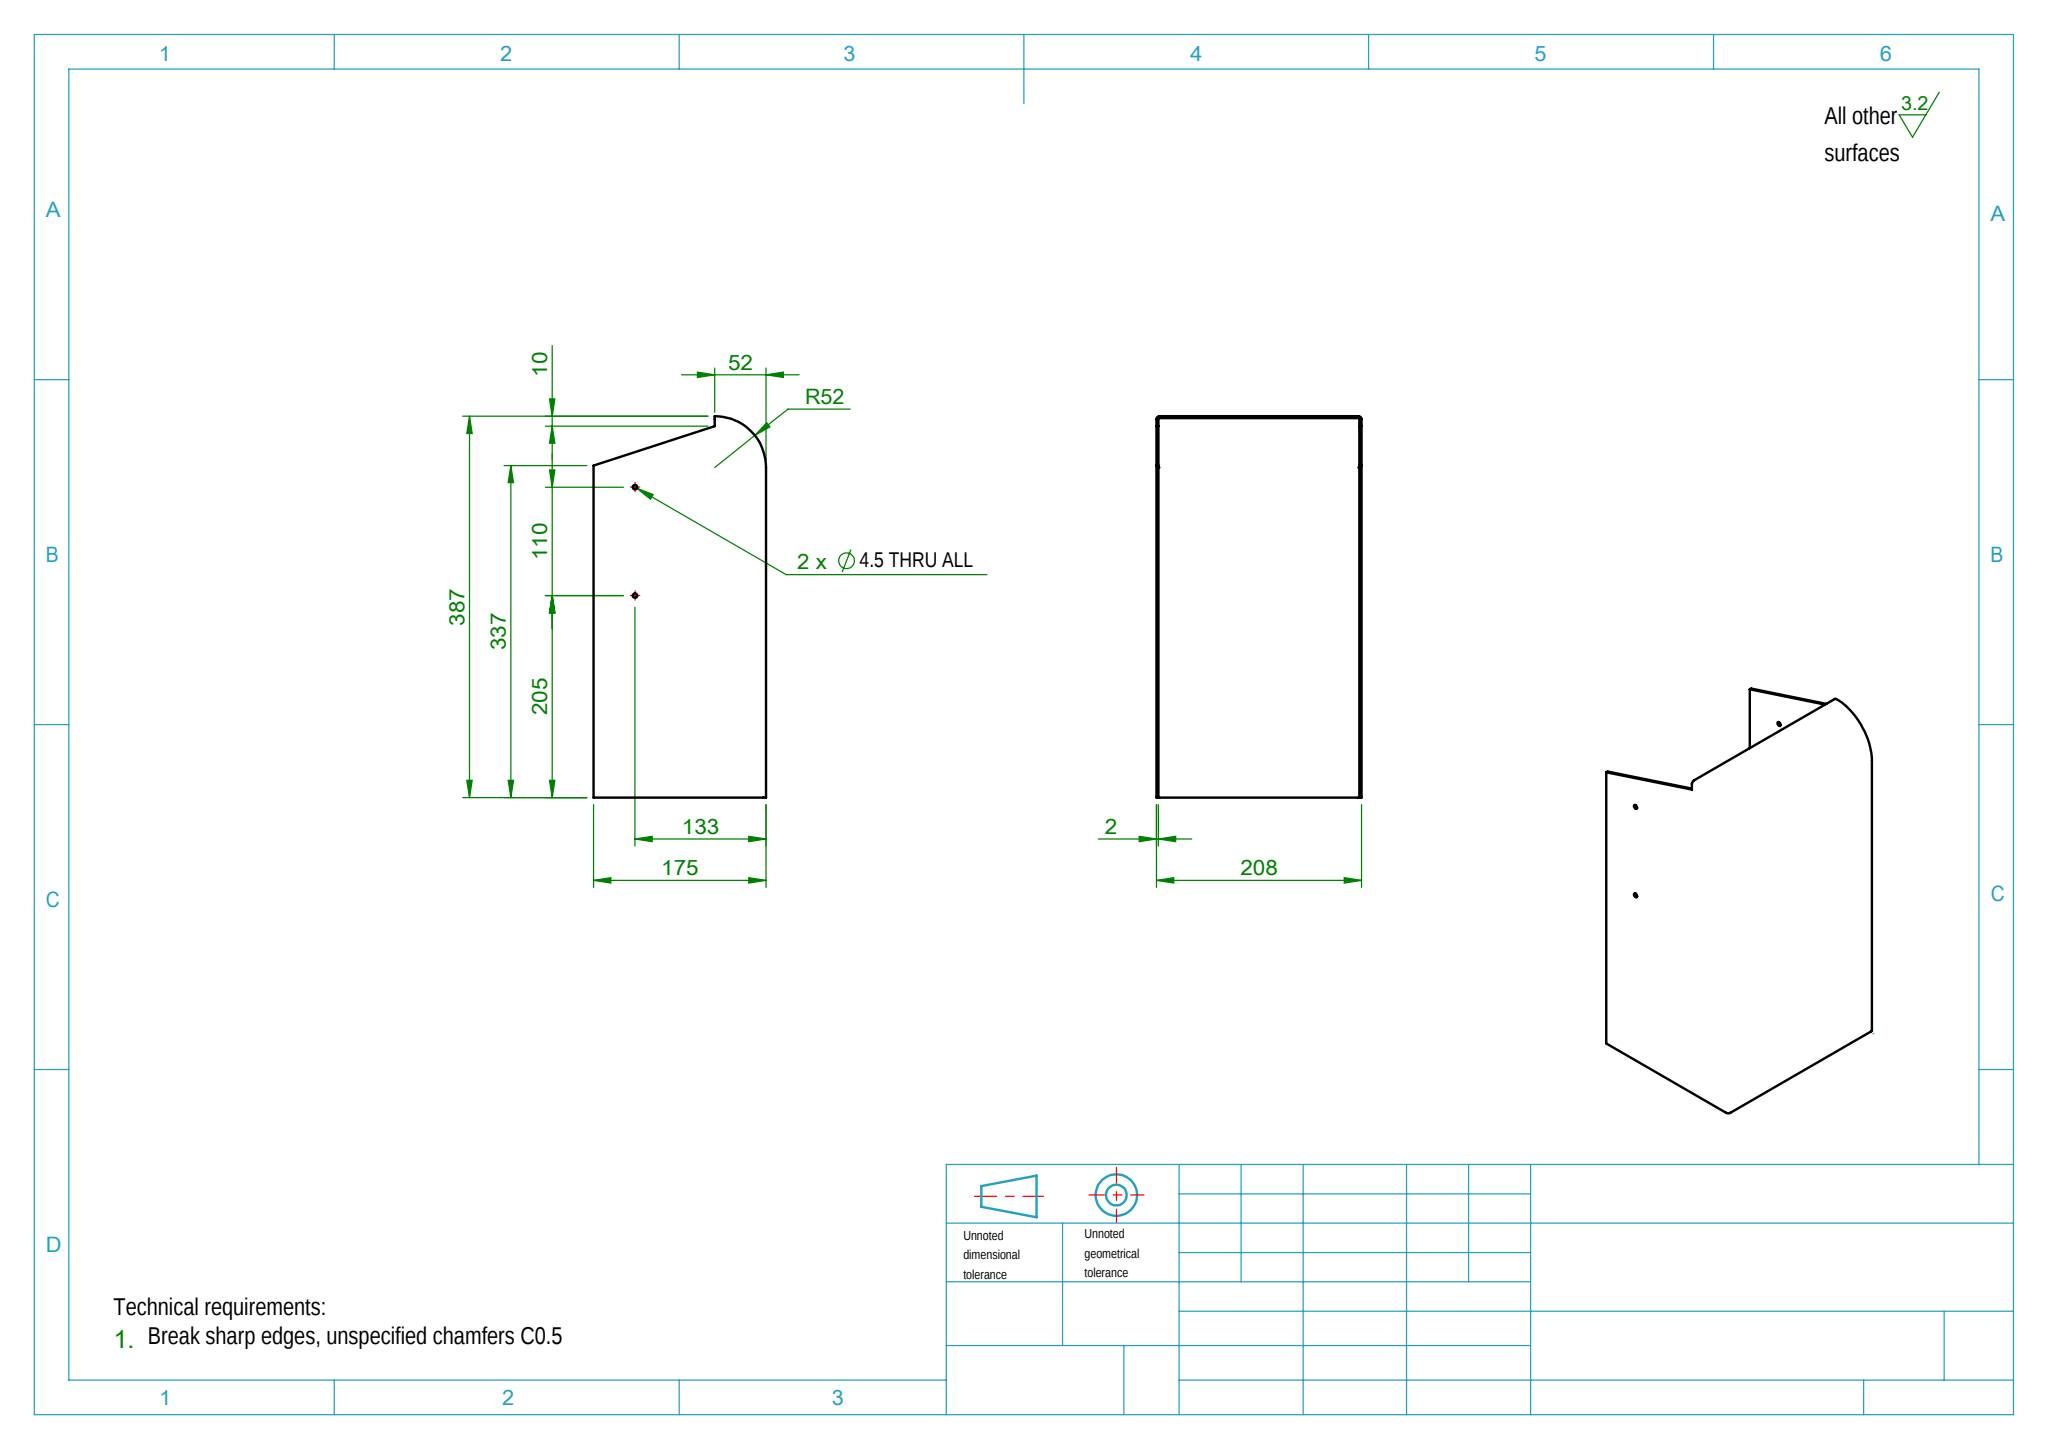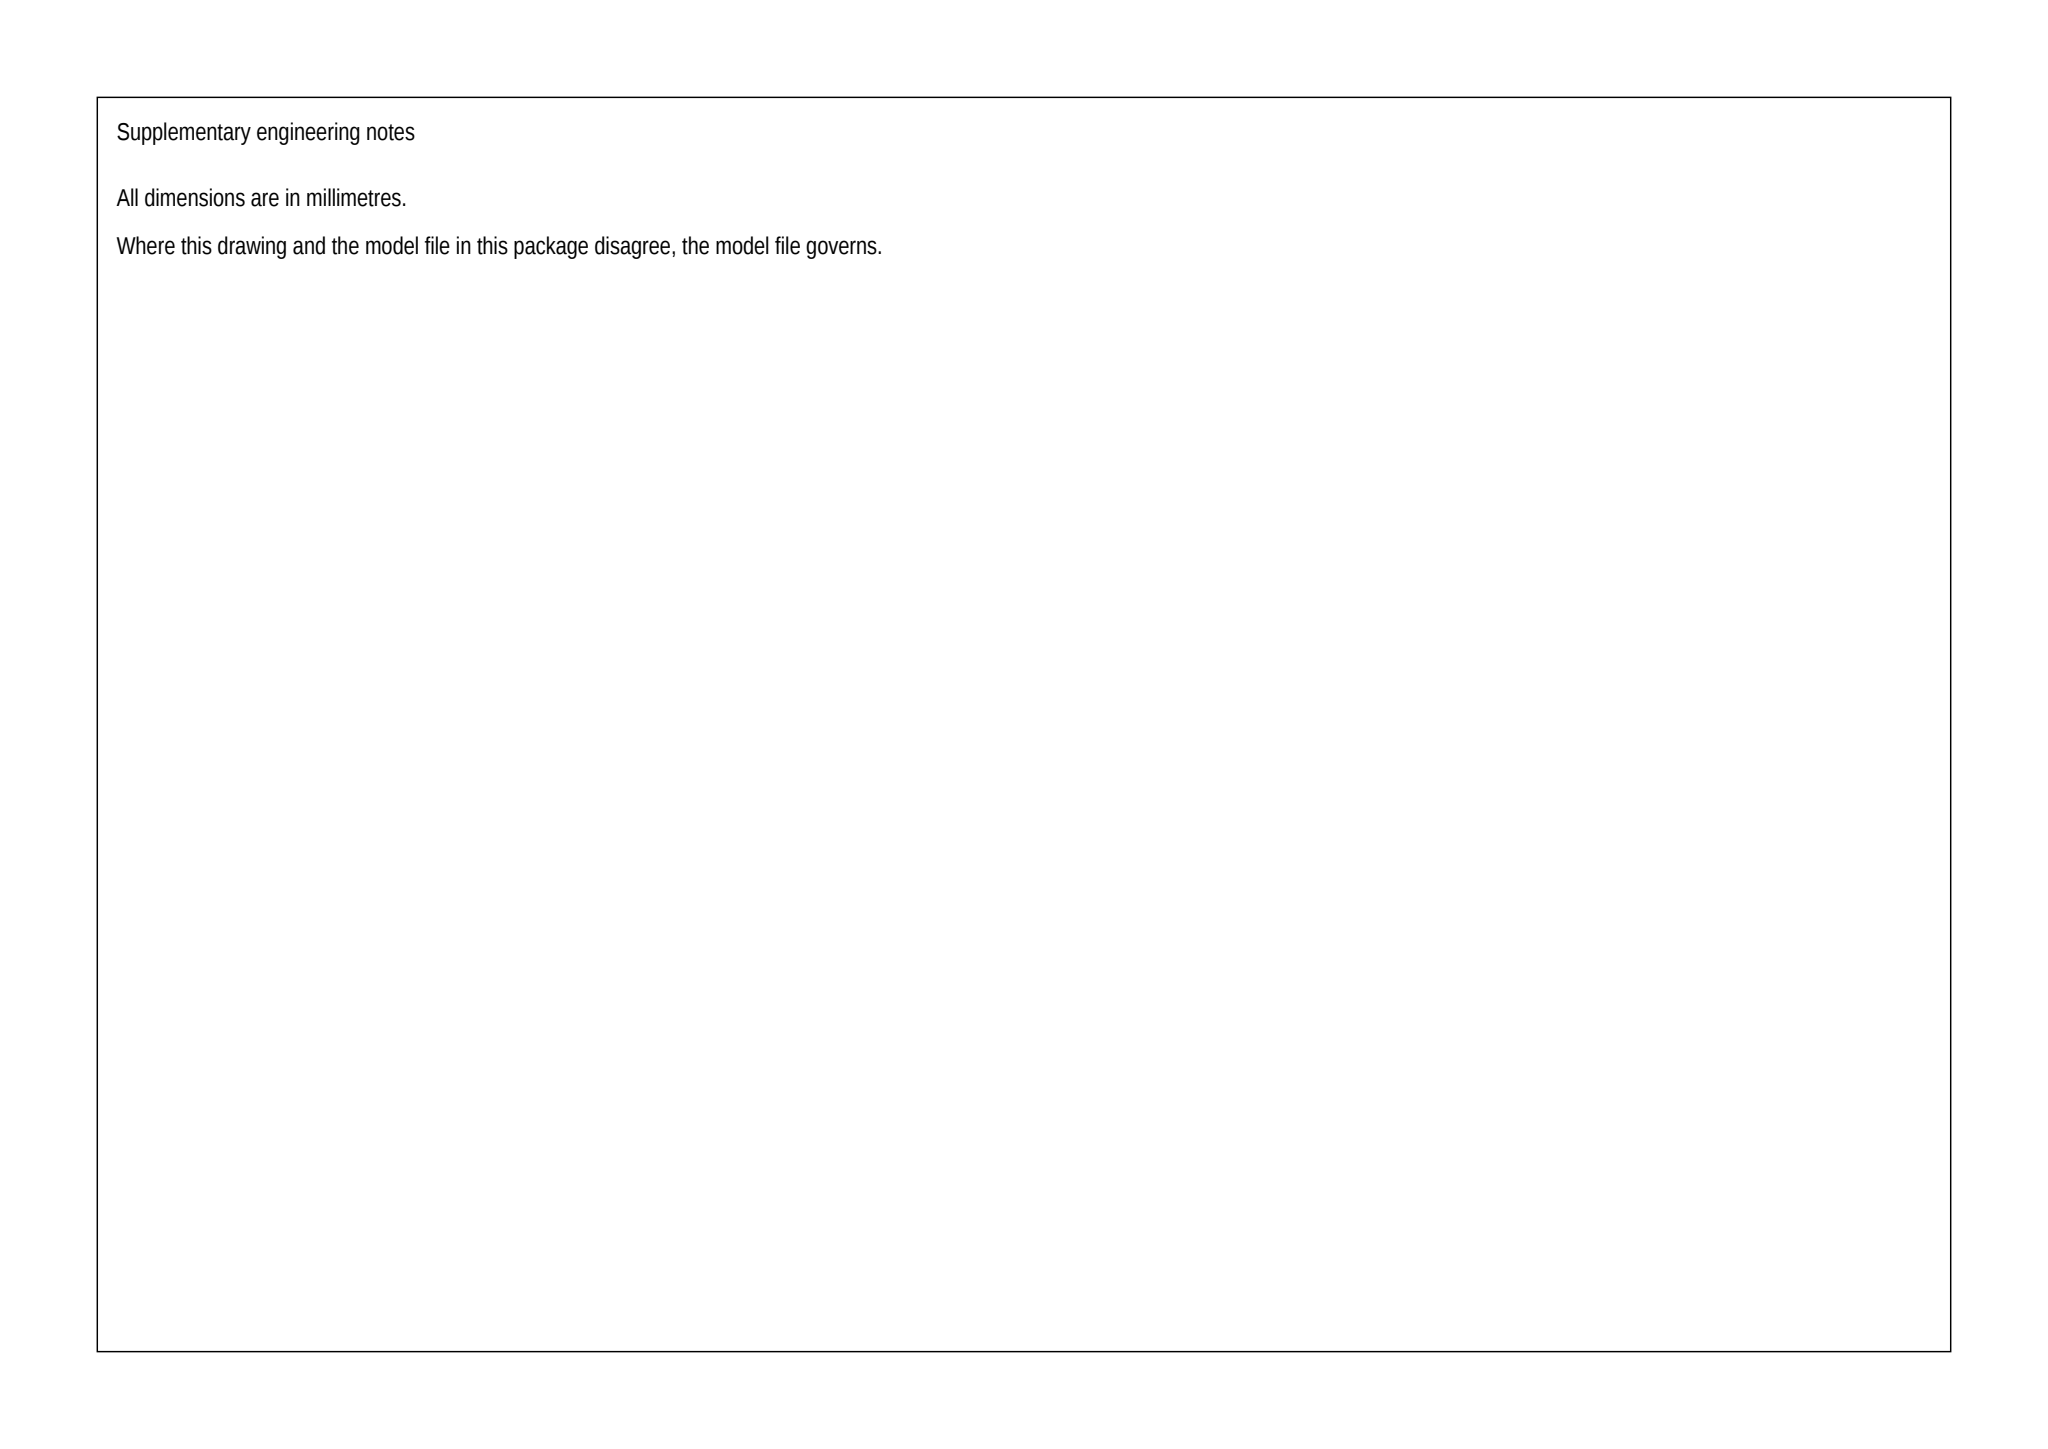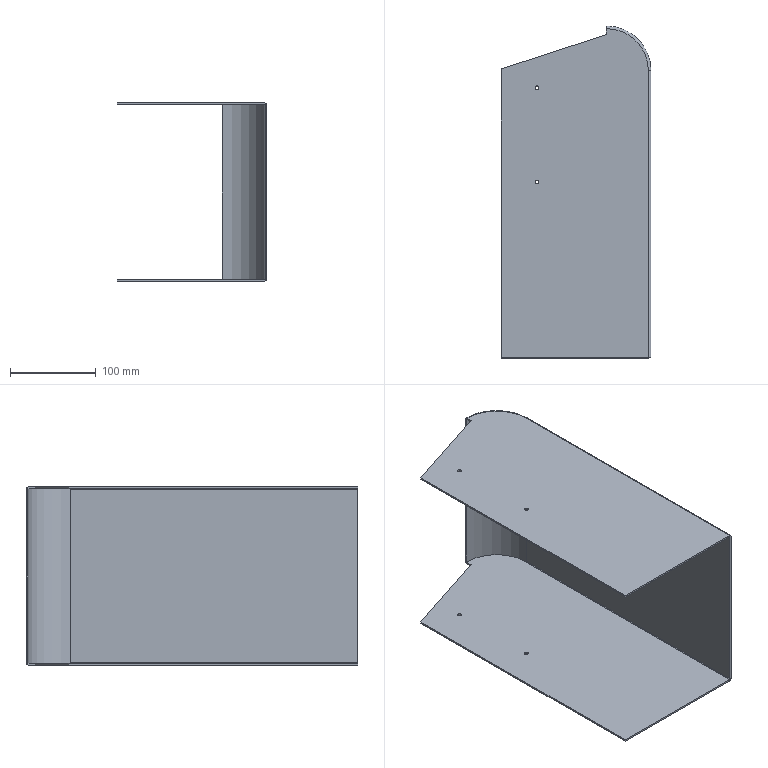Part | SolidWorks | mm | 1 solid | 34 faces | box 175 x 387 x 208 mm | volume 421595 mm3 | plane 18 | cylinder 14 | torus 2 | commonest cylinder face diameters 4.5 x8 6 x2 2 x2 104 x1 100 x1
Drawing notes:
SIDE & RETURN PANELS 335 HIGH FROM BOTTOM EDGE | from the solid: y-planes at 0 and 335 (2 faces); bend cyls Ø2/Ø6 axis y, length 335
RETURN PANEL 173 WIDE FROM 2ND BEND CL | from the solid: x-planes at 0 and 173; 2nd bend axis at x=172
2 BENDS 90°, INSIDE R1, OUTSIDE R3 (2 THK) | from the solid: Planes x=173/175 normal to z=0/2; bend cyls axis y at (x=172,z=3) and (x=172,z=205): Ø2 inner R1, Ø6 outer R3; fillet_radii 3.0 x2
2 x Ø4.5 THRU IN LINE, 133 FROM RH EDGE TYP | from the solid: Ø4.5 holes at x=42, y=205 and x=42, y=315; RH face x=175 → 175-42=133 both holes
RETURN FLANGE: 52 WIDE FROM RH EDGE (50 FROM BEND CL), 2 THK | from the solid: x-planes at 123 (flange free edge), 173 (bend CL), 175 (RH outer face); 175-123=52, 173-123=50; flange thk = 2 (z-planes 0/2)